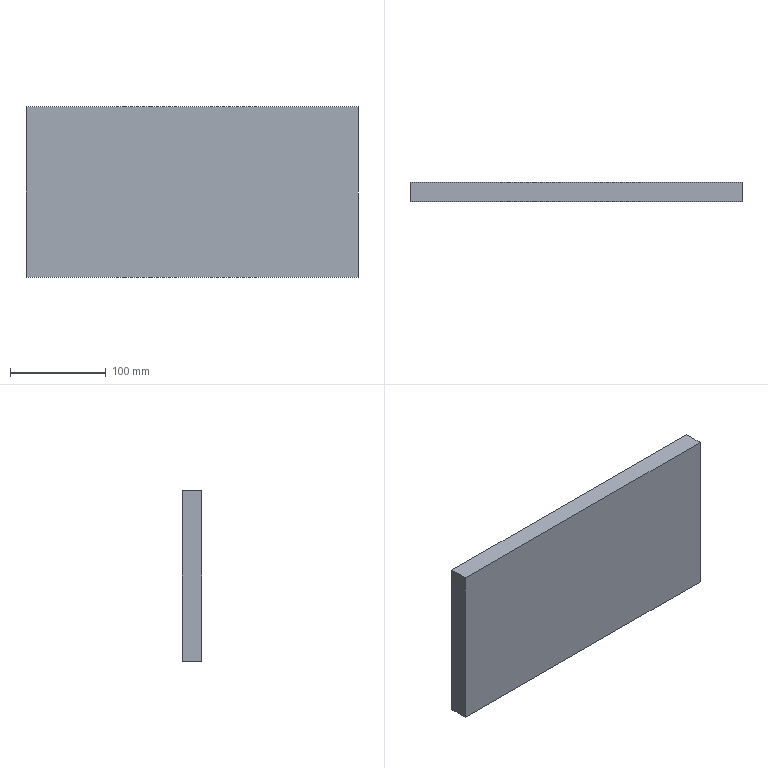Component | SolidWorks | 100-07-1 | 1 solid | 6 faces | box 346 x 20 x 178 mm | volume 1231760 mm3 | plane 6 | material 45
build123d program:
from build123d import *

# Parameters (mm, degrees)
SKETCH1_W           = 178
SKETCH1_H           = 346
BOSS_EXTRUDE1_DEPTH = 10


with BuildPart() as part:
    # Sketch1 → Boss-Extrude1 (new, symmetric)
    with BuildSketch(Plane(origin=(0, 0, 0), x_dir=(1, 0, 0), z_dir=(0, 1, 0))):
        Rectangle(SKETCH1_W, SKETCH1_H)
    extrude(amount=BOSS_EXTRUDE1_DEPTH, both=True)


solid = part.part

# Placed as in the assembly
solid = solid.moved(Location((-127, 284, 0), (0, 90, 0)))
STEP:
#1=COLOUR_RGB('',0.7922,0.8196,0.9333);
#2=FILL_AREA_STYLE_COLOUR('',#1);
#3=FILL_AREA_STYLE('',(#2));
#4=SURFACE_STYLE_FILL_AREA(#3);
#5=SURFACE_SIDE_STYLE('',(#4));
#6=SURFACE_STYLE_USAGE(.BOTH.,#5);
#7=PRESENTATION_STYLE_ASSIGNMENT((#6));
#8=CARTESIAN_POINT('',(1.811,10.787,-3.504));
#9=VERTEX_POINT('',#8);
#10=CARTESIAN_POINT('',(-11.811,10.787,-3.504));
#11=VERTEX_POINT('',#10);
#12=CARTESIAN_POINT('',(-11.811,10.787,-3.504));
#13=DIRECTION('',(-1.,0.,-0.));
#14=VECTOR('',#13,39.37);
#15=LINE('',#12,#14);
#16=EDGE_CURVE('',#9,#11,#15,.T.);
#17=ORIENTED_EDGE('',*,*,#16,.T.);
#18=CARTESIAN_POINT('',(-11.811,11.575,-3.504));
#19=VERTEX_POINT('',#18);
#20=CARTESIAN_POINT('',(-11.811,11.575,-3.504));
#21=DIRECTION('',(-0.,-1.,0.));
#22=VECTOR('',#21,39.37);
#23=LINE('',#20,#22);
#24=EDGE_CURVE('',#19,#11,#23,.T.);
#25=ORIENTED_EDGE('',*,*,#24,.F.);
#26=CARTESIAN_POINT('',(1.811,11.575,-3.504));
#27=VERTEX_POINT('',#26);
#28=CARTESIAN_POINT('',(-11.811,11.575,-3.504));
#29=DIRECTION('',(-1.,0.,-0.));
#30=VECTOR('',#29,39.37);
#31=LINE('',#28,#30);
#32=EDGE_CURVE('',#27,#19,#31,.T.);
#33=ORIENTED_EDGE('',*,*,#32,.F.);
#34=CARTESIAN_POINT('',(1.811,11.575,-3.504));
#35=DIRECTION('',(-0.,-1.,0.));
#36=VECTOR('',#35,39.37);
#37=LINE('',#34,#36);
#38=EDGE_CURVE('',#27,#9,#37,.T.);
#39=ORIENTED_EDGE('',*,*,#38,.T.);
#40=EDGE_LOOP('',(#17,#25,#33,#39));
#41=FACE_OUTER_BOUND('',#40,.T.);
#42=CARTESIAN_POINT('',(-11.811,11.575,-3.504));
#43=DIRECTION('',(-0.,0.,1.));
#44=DIRECTION('',(1.,-0.,0.));
#45=AXIS2_PLACEMENT_3D('',#42,#43,#44);
#46=PLANE('',#45);
#47=ADVANCED_FACE('',(#41),#46,.F.);
#48=CARTESIAN_POINT('',(-11.811,10.787,3.504));
#49=VERTEX_POINT('',#48);
#50=CARTESIAN_POINT('',(-11.811,10.787,3.504));
#51=DIRECTION('',(-0.,0.,1.));
#52=VECTOR('',#51,39.37);
#53=LINE('',#50,#52);
#54=EDGE_CURVE('',#11,#49,#53,.T.);
#55=ORIENTED_EDGE('',*,*,#54,.T.);
#56=CARTESIAN_POINT('',(-11.811,11.575,3.504));
#57=VERTEX_POINT('',#56);
#58=CARTESIAN_POINT('',(-11.811,11.575,3.504));
#59=DIRECTION('',(-0.,-1.,0.));
#60=VECTOR('',#59,39.37);
#61=LINE('',#58,#60);
#62=EDGE_CURVE('',#57,#49,#61,.T.);
#63=ORIENTED_EDGE('',*,*,#62,.F.);
#64=CARTESIAN_POINT('',(-11.811,11.575,3.504));
#65=DIRECTION('',(-0.,0.,1.));
#66=VECTOR('',#65,39.37);
#67=LINE('',#64,#66);
#68=EDGE_CURVE('',#19,#57,#67,.T.);
#69=ORIENTED_EDGE('',*,*,#68,.F.);
#70=ORIENTED_EDGE('',*,*,#24,.T.);
#71=EDGE_LOOP('',(#55,#63,#69,#70));
#72=FACE_OUTER_BOUND('',#71,.T.);
#73=CARTESIAN_POINT('',(-11.811,11.575,3.504));
#74=DIRECTION('',(1.,-0.,0.));
#75=DIRECTION('',(0.,-0.,-1.));
#76=AXIS2_PLACEMENT_3D('',#73,#74,#75);
#77=PLANE('',#76);
#78=ADVANCED_FACE('',(#72),#77,.F.);
#79=CARTESIAN_POINT('',(1.811,10.787,3.504));
#80=VERTEX_POINT('',#79);
#81=CARTESIAN_POINT('',(-11.811,10.787,3.504));
#82=DIRECTION('',(1.,-0.,0.));
#83=VECTOR('',#82,39.37);
#84=LINE('',#81,#83);
#85=EDGE_CURVE('',#49,#80,#84,.T.);
#86=ORIENTED_EDGE('',*,*,#85,.T.);
#87=CARTESIAN_POINT('',(1.811,11.575,3.504));
#88=VERTEX_POINT('',#87);
#89=CARTESIAN_POINT('',(1.811,11.575,3.504));
#90=DIRECTION('',(-0.,-1.,0.));
#91=VECTOR('',#90,39.37);
#92=LINE('',#89,#91);
#93=EDGE_CURVE('',#88,#80,#92,.T.);
#94=ORIENTED_EDGE('',*,*,#93,.F.);
#95=CARTESIAN_POINT('',(-11.811,11.575,3.504));
#96=DIRECTION('',(1.,-0.,0.));
#97=VECTOR('',#96,39.37);
#98=LINE('',#95,#97);
#99=EDGE_CURVE('',#57,#88,#98,.T.);
#100=ORIENTED_EDGE('',*,*,#99,.F.);
#101=ORIENTED_EDGE('',*,*,#62,.T.);
#102=EDGE_LOOP('',(#86,#94,#100,#101));
#103=FACE_OUTER_BOUND('',#102,.T.);
#104=CARTESIAN_POINT('',(-11.811,11.575,3.504));
#105=DIRECTION('',(0.,-0.,-1.));
#106=DIRECTION('',(-1.,0.,-0.));
#107=AXIS2_PLACEMENT_3D('',#104,#105,#106);
#108=PLANE('',#107);
#109=ADVANCED_FACE('',(#103),#108,.F.);
#110=CARTESIAN_POINT('',(1.811,10.787,3.504));
#111=DIRECTION('',(0.,-0.,-1.));
#112=VECTOR('',#111,39.37);
#113=LINE('',#110,#112);
#114=EDGE_CURVE('',#80,#9,#113,.T.);
#115=ORIENTED_EDGE('',*,*,#114,.T.);
#116=ORIENTED_EDGE('',*,*,#38,.F.);
#117=CARTESIAN_POINT('',(1.811,11.575,3.504));
#118=DIRECTION('',(0.,-0.,-1.));
#119=VECTOR('',#118,39.37);
#120=LINE('',#117,#119);
#121=EDGE_CURVE('',#88,#27,#120,.T.);
#122=ORIENTED_EDGE('',*,*,#121,.F.);
#123=ORIENTED_EDGE('',*,*,#93,.T.);
#124=EDGE_LOOP('',(#115,#116,#122,#123));
#125=FACE_OUTER_BOUND('',#124,.T.);
#126=CARTESIAN_POINT('',(1.811,11.575,3.504));
#127=DIRECTION('',(-1.,0.,-0.));
#128=DIRECTION('',(-0.,0.,1.));
#129=AXIS2_PLACEMENT_3D('',#126,#127,#128);
#130=PLANE('',#129);
#131=ADVANCED_FACE('',(#125),#130,.F.);
#132=ORIENTED_EDGE('',*,*,#32,.T.);
#133=ORIENTED_EDGE('',*,*,#68,.T.);
#134=ORIENTED_EDGE('',*,*,#99,.T.);
#135=ORIENTED_EDGE('',*,*,#121,.T.);
#136=EDGE_LOOP('',(#132,#133,#134,#135));
#137=FACE_OUTER_BOUND('',#136,.T.);
#138=CARTESIAN_POINT('',(-5.,11.575,0.));
#139=DIRECTION('',(0.,1.,-0.));
#140=DIRECTION('',(-1.,0.,-0.));
#141=AXIS2_PLACEMENT_3D('',#138,#139,#140);
#142=PLANE('',#141);
#143=ADVANCED_FACE('',(#137),#142,.T.);
#144=ORIENTED_EDGE('',*,*,#16,.F.);
#145=ORIENTED_EDGE('',*,*,#114,.F.);
#146=ORIENTED_EDGE('',*,*,#85,.F.);
#147=ORIENTED_EDGE('',*,*,#54,.F.);
#148=EDGE_LOOP('',(#144,#145,#146,#147));
#149=FACE_OUTER_BOUND('',#148,.T.);
#150=CARTESIAN_POINT('',(-5.,10.787,0.));
#151=DIRECTION('',(0.,1.,-0.));
#152=DIRECTION('',(-1.,0.,-0.));
#153=AXIS2_PLACEMENT_3D('',#150,#151,#152);
#154=PLANE('',#153);
#155=ADVANCED_FACE('',(#149),#154,.F.);
#156=CLOSED_SHELL('',(#47,#78,#109,#131,#143,#155));
#157=MANIFOLD_SOLID_BREP('',#156);
#158=STYLED_ITEM('',(#7),#157);
#159=(LENGTH_UNIT()NAMED_UNIT(*)SI_UNIT($,.METRE.));
#160=LENGTH_MEASURE_WITH_UNIT(LENGTH_MEASURE(0.0254),#159);
#161=DIMENSIONAL_EXPONENTS(1.,0.,0.,0.,0.,0.,0.);
#162=(CONVERSION_BASED_UNIT('',#160)LENGTH_UNIT()NAMED_UNIT(#161));
#163=UNCERTAINTY_MEASURE_WITH_UNIT(LENGTH_MEASURE(0.00001),#162,'','');
#164=(NAMED_UNIT(*)PLANE_ANGLE_UNIT()SI_UNIT($,.RADIAN.));
#165=(NAMED_UNIT(*)SI_UNIT($,.STERADIAN.)SOLID_ANGLE_UNIT());
#166=(GEOMETRIC_REPRESENTATION_CONTEXT(3)GLOBAL_UNCERTAINTY_ASSIGNED_CONTEXT((#163))GLOBAL_UNIT_ASSIGNED_CONTEXT((#162,#164,#165))REPRESENTATION_CONTEXT('',''));
#167=MECHANICAL_DESIGN_GEOMETRIC_PRESENTATION_REPRESENTATION('',(#158),#166);
#168=PRESENTATION_LAYER_ASSIGNMENT('','',(#158));
#169=CARTESIAN_POINT('',(0.,0.,0.));
#170=DIRECTION('',(0.,0.,1.));
#171=DIRECTION('',(1.,0.,0.));
#172=AXIS2_PLACEMENT_3D('',#169,#170,#171);
#173=(LENGTH_UNIT()NAMED_UNIT(*)SI_UNIT($,.METRE.));
#174=LENGTH_MEASURE_WITH_UNIT(LENGTH_MEASURE(0.0254),#173);
#175=DIMENSIONAL_EXPONENTS(1.,0.,0.,0.,0.,0.,0.);
#176=(CONVERSION_BASED_UNIT('',#174)LENGTH_UNIT()NAMED_UNIT(#175));
#177=UNCERTAINTY_MEASURE_WITH_UNIT(LENGTH_MEASURE(0.00001),#176,'','');
#178=(NAMED_UNIT(*)PLANE_ANGLE_UNIT()SI_UNIT($,.RADIAN.));
#179=(NAMED_UNIT(*)SI_UNIT($,.STERADIAN.)SOLID_ANGLE_UNIT());
#180=(GEOMETRIC_REPRESENTATION_CONTEXT(3)GLOBAL_UNCERTAINTY_ASSIGNED_CONTEXT((#177))GLOBAL_UNIT_ASSIGNED_CONTEXT((#176,#178,#179))REPRESENTATION_CONTEXT('',''));
#181=ADVANCED_BREP_SHAPE_REPRESENTATION('',(#157,#172),#180);